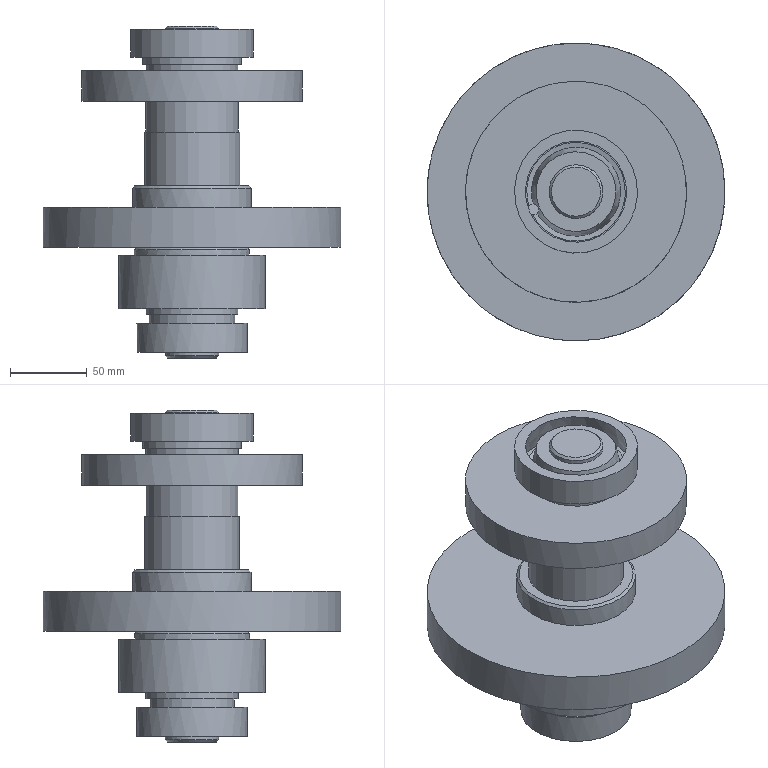Assembly | NX | mm | 9 component files | 13 solids | 169 faces | box 193.75 x 193.75 x 216 mm | volume 1750767 mm3 | plane 105 | cylinder 52 | cone 12 | commonest cylinder face diameters 45 x24 35 x6 60 x3 55.587 x3 64.269 x3 33 x2 193.75 x1 77.253 x1
Bill of materials:
unnamed part 1 | 1 |  | Flat circular disc with a smaller coaxial cylindrical hub on one side and a through bore with six rectangular notches (spline-like) around it.
unnamed part 2 | 1 |  | Stepped cylindrical shaft with a longer, larger central section carrying six longitudinal rectangular ridges (spline-like) and plain smaller-diameter cylindrical ends.
unnamed part 3 | 1 |  | Annular body made of concentric outer and inner rings separated by an open annular gap. A single small rounded element sits in the gap. The outer profile is stepped, with a narrower lower step.
unnamed part 4 | 2 |  | Thin flat annular ring (washer-like) with a plain circular central hole.
unnamed part 5 | 1 |  | Flat circular disc with a short raised, chamfered coaxial hub on one face and a through bore with six rectangular notches.
unnamed part 6 | 1 |  | Thick cylindrical ring with a slightly smaller, chamfered raised step on one face and a large through bore with six rectangular notches.
unnamed part 7 | 1 |  | Annular body with an outer ring and a concentric inner ring that sticks out above the outer ring, separated by a narrow annular gap. A small rounded element is visible at one point in the gap.
unnamed part 8 | 1 |  | Thin-walled plain cylindrical tube or sleeve with a uniform circular cross-section.
Mates:
1. touch align | zhouV3 1 face | zhouV1 1 face
2. touch align | zhouV4 1 face | zhouV1 1 face
3. parallel | zhouV1 1 face | zhouV4 1 face
4. distance | zhouV1 1 face | zhouV4 1 face
5. parallel | zhouV2 1 face | zhouV1 1 face
6. touch align | zhouV2 1 face | zhouV1 1 face
7. touch align | zhouV2 1 face | zhouV4 1 face
8. touch align | ct-zhou5-zhoucheng2 1 face | zhouV1 1 face
9. touch align | ct-zhou5-taotong1 1 face | zhouV3 1
10. touch align | ct-zhou5-dangquan1 2 face | zhouV3 1 face
11. touch align | zhouV3 1 face | ct-zhou5-dangquan1 2 face
12. touch align | ct-zhou5-zhoucheng2 1 face | ct-zhou5-dangquan1 2 face
13. touch align | ct-zhou5-taotong1 1 face | zhouV2 1 face
14. touch align | zhouV3 1 | ct-zhou5-taotong1 1 face
15. touch align | ct-zhou5-dangquan1 1 face | zhouV1 1 face
16. touch align | ct-zhou5-dangquan1 1 face | zhouV4 1 face
17. touch align | ct-zhou5-zhoucheng1 1 face | ct-zhou5-dangquan1 1 face